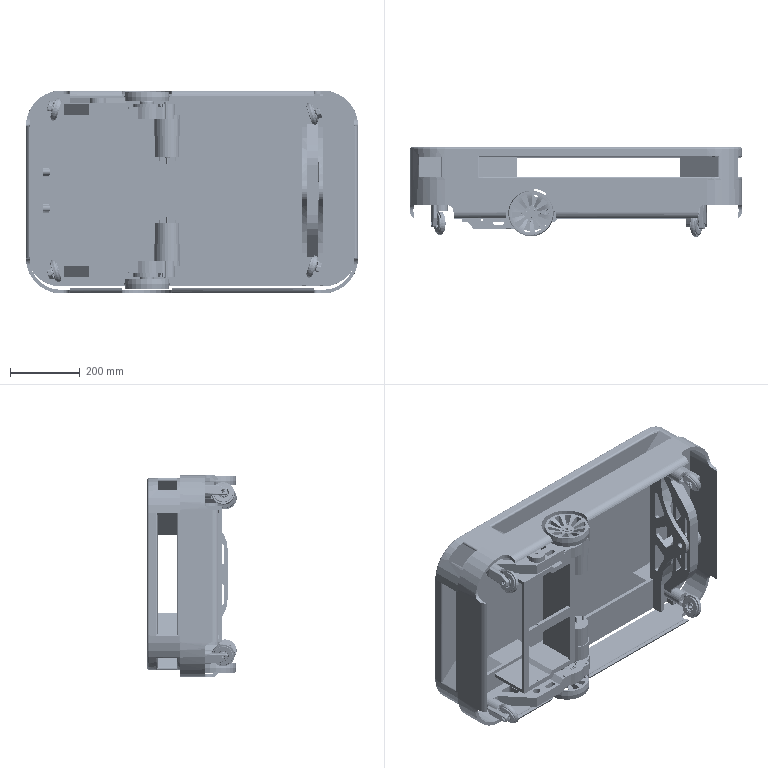Assembly | SolidWorks | mm | 60 component files | 355 solids | 6056 faces | box 950 x 255.66 x 580 mm | volume 29114725 mm3 | cylinder 3134 | plane 1494 | sphere 690 | torus 552 | cone 146 | spline 40 | commonest cylinder face diameters 1 x268 6.975 x266 0.6 x260 6.15 x192 23.75 x168 21.25 x168 4 x162 10 x133
Bill of materials:
Bracket1 | 1 |  | Elongated stepped bracket/plate. At one end is a rounded eye with a hexagonal hole. A triangular cutout and rectangular, round and slotted openings run along the body. At the other end is a large circular bore with a counterbored/recessed seat, an adjacent smaller round hole, and several small holes around both bores.
BrushedDCMotor | 1 |  | Cylindrical body with two diameters. A stepped shaft protrudes from one end face, which has a raised boss. A small offset feature and pin-like protrusions are at the opposite end.
DriveWheel | 1 |  | Wheel-like disc, or rim, with a flanged outer rim and twelve tapered radial spokes. The central hub opening has semicircular notches around it.
DriveWheelRubber | 1 | Natural Rubber | Thin-walled cylindrical ring or band with a short axial length relative to its diameter. The outer surface appears slightly crowned or faceted.
FlatWasher | 1 |  | Flat annular disc with a central circular hole: a plain washer-like shape.
Gasket | 4 |  | Flat open ring with a gap. Each end has a lug with a small hole. The shape resembles an internal-style retaining ring, with the lugs on the inner side.
GB_T276-2013[DeepGrooveBallBearing[60000]608] | 1 | AISI 304 | Annular assembly-like body: concentric outer and inner rings separated by a gap, with a central bore. The edges are rounded.
Gb_t276-2013[DeepGrooveBallBearing[60000]61908] | 2 |  | Thin-section annular body with concentric outer and inner rings, a narrow gap between them, and a large bore relative to its outer diameter.
GB_T276-2013[DeepGrooveBallBearing[60000]6300] | 7 | AISI 304 | Annular body with concentric outer and inner rings, an annular gap, and a relatively small central bore.
GuideWheelBracket | 2 |  | Arm or bracket with a cylindrical sleeve (a through-bore collar) at one end. A tapered flat lever extends from the sleeve to a rounded tip, which has a countersunk or counterbored small hole.
GuideWheelHub | 2 |  | Grooved ring, like a pulley or grommet: an annular body with a concave groove around its outside between two flanges, and a central bore with an internal step.
GuideWheelRubber | 2 |  | Annular ring with a roughly rectangular cross-section and slightly rounded edges. The section is thicker radially than the thin band part.
LargeGear | 1 |  | Compound spur-gear part: a thin wide toothed disc with a tall cylindrical hub on one face. A smaller lobed boss with six rounded lobes sits on top of the hub, and a small round bore runs through the center.
ProtectivePlate | 1 |  | Flat plate with a large circular through-opening and a smaller circular through-opening beside it. The outline is mostly rectangular, with arc-shaped bulges around both openings. There are four small corner holes, and part of the plate is a thicker raised region.
SmallGear | 1 |  | Spur gear with a short raised collar on one face. Its central bore is D-shaped, with one flat side.
DeepGrooveBallBearing[60000][61900] | 1 | AISI 304 | Ring assembly with concentric inner and outer rings and a visible annular gap between them, in a form that looks like a bearing. It is relatively wide compared with the ring cross-section.
GuideWheelBracket2 | 1 |  | Elongated bracket link with a curved, offset body. Each end has a rounded eye with a hexagonal hole. The central web has triangular and slot-shaped lightening cutouts arranged like a truss around a small round hole.
MirrorGasket | 4 |  | Thin flat open ring with a gap. Each end of the opening has a lug with a small round hole. The overall form resembles a retaining ring.
MirrorGB_T276-2013[DeepGrooveBallBearing[60000]6300] | 7 | AISI 304 | Ring assembly with concentric inner and outer rings and an annular gap between them, in a form that looks like a bearing. It has a smaller bore relative to its outer diameter than unnamed part.
MirrorGuideWheelBracket | 2 |  | Clamp-like arm: a cylindrical collar with a large bore, with a lever arm extending from one side. Near the end of the arm is a small round hole with a hexagonal recess.
MirrorGuideWheelHub | 2 |  | Grooved wheel or pulley-like ring: an annular body with a concave groove running around its outer edge between two flanges, and a large central bore.
MirrorGuideWheelRubber | 2 |  | Plain ring with a roughly rectangular cross-section, rounded or slightly chamfered edges, and a large inner diameter compared with its wall thickness.
MirrorBracket1 | 1 |  | Mounting-plate bracket with an irregular outline and a stepped thickness. It has a large circular opening and a smaller circular opening ringed by a pattern of small holes. There are also rectangular slots, a round hole, a triangular cutout, and an end eye with a hexagonal hole.
MirrorBrushedDCMotor | 1 |  | Cylindrical body made of two coaxial sections of slightly different diameters. One end has a small central shaft and two flat tab-like protrusions. The other end has an off-center smaller cylindrical boss and a stepped output shaft. The form resembles a geared-motor housing.
MirrorDriveWheel | 1 |  | Spoked wheel or spool-like disc. A circular body has twelve tapered spoke windows, a central bore with semicircular notches around it, and a raised flange at each axial end with a shallow recessed band between them.
MirrorDriveWheelRubber | 1 | Natural Rubber | Short thin-walled cylindrical ring (band) with an open bore and a small radial wall thickness. The outer surface has a slight break or taper at mid-height.
MirrorFlatWasher | 1 |  | Flat annular disc (washer-like) with one concentric through-hole and uniform thickness.
MirrorGB_T276-2013[DeepGrooveBallBearing[60000]608] | 1 | AISI 304 | Group of concentric rings: an outer ring and an inner ring with a central bore, separated by an annular gap that holds a thinner intermediate ring. The edges are rounded. The overall form looks like a bearing.
Mirrorgb_t276-2013[DeepGrooveBallBearing[60000]61908] | 2 |  | Thin-section set of concentric rings: an outer ring and an inner ring with a large bore, separated by a narrow gap. The edges are rounded. The form looks like a thin-section bearing.
MirrorGuardPlate | 1 |  | Stepped mounting plate (flange). It has a large circular through-opening with an internal step, a side lobe with a smaller stepped circular opening, and four corner through-holes in a rectangular plate region with rounded corners.
MirrorLargeGear | 1 |  | Compound spur gear part: a large spur gear ring around a tall cylindrical hub, with a smaller toothed pinion section at one end. There is a hexagonal recess at the top of the hub and a small round axial hole.
MirrorSmallGear | 1 |  | Spur gear with straight teeth, a central bore that appears to have one flat (D-shaped), and a short smaller-diameter hub shoulder on one face.
Part27 | 1 |  | Thin-walled rounded-rectangle frame (open band) with no top or bottom face. It has a semicircular notch in the edge of each long side and rectangular relief notches near the corners.
Tray | 1 |  | Complex shallow housing or tray: a rounded-rectangle body with a flat face plate, an internal perimeter frame and ribs, a box-like compartment near one end, curved slotted arm features near the other end, and small pins or tabs on the face.
Mates:
1. parallel | FrontGuideWheel-1/GuideWheelBracket2-1 face at (544.259, 72.387, -327.387) dir (0, 1, 0) | Tray-2 face at (-191.241, 138, -41.572) dir (0, -1, 0)
2. width | FrontGuideWheel-1/GuideWheelBracket2-1 face at (544.259, 87.387, -288.413) dir (1, 0, 0) | FrontGuideWheel-1/GuideWheelBracket2-1 face at (513.259, 87.387, -288.413) dir (-1, 0, 0) | Tray-2 face at (545.759, 3.167, 58.428) dir (-1, 0, 0) | Tray-2 face at (511.759, 3.167, 58.428) dir (1, 0, 0)
3. parallel | DriveDevice-1/Bracket1-1 face at (0, 0, 31) dir (0, 0, 1) | Tray-2 face at (558.759, 232, 58.428) dir (0, 0, 1)
4. distance | DriveDevice-1/Bracket1-1 face at (0, 118, 31) dir (0, 1, 0) | Tray-2 face at (-191.241, 138, -41.572) dir (0, -1, 0)
5. concentric | FrontGuideWheel-1/DeepGrooveBallBearing[60000][61900]-1 edge at (544.559, 27.686, -216.572) dir (-1, 0, 0) r 5.3 | Tray-2 edge at (558.759, 27.686, -216.572) dir (1, 0, 0) r 8.309
6. width | Tray-2 face at (498.759, 110, -486.572) dir (-1, 0, 0) | Tray-2 face at (558.759, 110, -486.572) dir (1, 0, 0) | FrontGuideWheel-1/GuideWheelBracket2-1 face at (544.259, 87.387, -288.413) dir (1, 0, 0) | FrontGuideWheel-1/GuideWheelBracket2-1 face at (513.259, 87.387, -288.413) dir (-1, 0, 0)
7. coincident | Tray-2 face at (-191.241, 138, -41.572) dir (0, -1, 0) | Part27-1 face at (-191.241, 138, -411.572) dir (0, 1, 0)
8. coincident | Tray-2 face at (-291.241, 232, -41.572) dir (-1, 0, 0) | Part27-1 face at (-291.241, 28, -31.572) dir (-1, 0, 0)
9. coincident | Tray-2 face at (558.759, 232, 58.428) dir (0, 0, 1) | Part27-1 face at (558.759, 28, 58.428) dir (0, 0, -1)
10. concentric | Bracket1-1 edge at (55, 43, 2.5) dir (0, 0, -1) r 32.2 | Gb_t276-2013[DeepGrooveBallBearing[60000]61908]-1 edge at (55, 43, -9.9) dir (0, 0, 1) r 31
11. coincident | Bracket1-1 face at (55, 43, -10.5) dir (0, 0, 1) | Gb_t276-2013[DeepGrooveBallBearing[60000]61908]-1 face at (71.985, 68.212, -10.5) dir (0, 0, -1)
12. concentric | Gb_t276-2013[DeepGrooveBallBearing[60000]61908]-1 edge at (55, 43, 1.5) dir (0, 0, 1) r 20.6 | LargeGear-1 edge at (55, 43, -13) dir (0, 0, -1) r 18.8
13. coincident | Gb_t276-2013[DeepGrooveBallBearing[60000]61908]-1 face at (66.51, 60.085, 1.5) dir (0, 0, 1) | LargeGear-1 face at (55, 43, 1.5) dir (0, 0, -1)
14. concentric | LargeGear-1 edge at (55, 43, 37.5) dir (0, 0, 1) r 18.8 | Gb_t276-2013[DeepGrooveBallBearing[60000]61908]-2 edge at (55, 43, 27.5) dir (0, 0, 1) r 20.6
15. coincident | LargeGear-1 face at (55, 43, 15.5) dir (0, 0, 1) | Gb_t276-2013[DeepGrooveBallBearing[60000]61908]-2 face at (73.287, 67.285, 15.5) dir (0, 0, -1)
16. coincident | Bracket1-1 face at (0, 0, 2.5) dir (0, 0, 1) | SmallGear-1 face at (109.394, 58.688, 2.5) dir (0, 0, -1)
17. coincident | SmallGear-1 face at (110, 43, 14.5) dir (0, 0, 1) | GB_T276-2013[DeepGrooveBallBearing[60000]6300]-1 face at (117.32, 58.232, 14.5) dir (0, 0, -1)
18. concentric | LargeGear-1 edge at (55, 43, 37.5) dir (0, 0, 1) r 18.8 | ProtectivePlate-1 edge at (55, 43, 31.5) dir (0, 0, 1) r 30.2
19. coincident | Bracket1-1 face at (0, 0, 16.5) dir (0, 0, 1) | ProtectivePlate-1 face at (85.418, 8.541, 16.5) dir (0, 0, -1)
20. concentric | LargeGear-1 edge at (55, 43, 53.5) dir (0, 0, 1) r 4.3 | FlatWasher-1 edge at (55, 43, 53.5) dir (0, 0, -1) r 4.3
21. coincident | LargeGear-1 face at (55, 43, 53.5) dir (0, 0, 1) | FlatWasher-1 face at (55, 43, 53.5) dir (0, 0, -1)
22. concentric | LargeGear-1 edge at (55, 43, 53.5) dir (0, 0, 1) r 4.3 | DriveWheel-1 edge at (55, 43, 37.5) dir (0, 0, 1) r 62
23. coincident | LargeGear-1 face at (55, 43, 37.5) dir (0, 0, 1) | DriveWheel-1 face at (55, 43, 37.5) dir (0, 0, -1)
24. concentric | LargeGear-1 face at (58.449, 57.598, 52.5) dir (0, 0, -1) r 785.398 | DriveWheel-1 face at (58.449, 57.598, 37.5) dir (0, 0, 1) r 5.5
25. concentric | GB_T276-2013[DeepGrooveBallBearing[60000]6300]-2 edge at (-203.866, 70.2, 20) dir (0, -1, 0) r 13.933 | GB_T276-2013[DeepGrooveBallBearing[60000]6300]-3 edge at (-203.866, 70.2, 20) dir (0, 1, 0) r 5.6
26. coincident | GB_T276-2013[DeepGrooveBallBearing[60000]6300]-2 face at (-220.649, 70.2, 18.017) dir (0, -1, 0) | GB_T276-2013[DeepGrooveBallBearing[60000]6300]-3 face at (-186.966, 70.2, 20.101) dir (0, 1, 0)
27. concentric | GuideWheelHub-1 edge at (-210.9, 15, 15.884) dir (-0.9559, 0, 0.2937) r 14 | GB_T276-2013[DeepGrooveBallBearing[60000]6300]-4 edge at (-210.9, 15, 15.884) dir (0.9559, 0, -0.2937) r 16.9
28. parallel | SmallGear-1 face at (115.607, 45.136, 30.54) dir (-0.9875, 0.1577, 0) | BrushedDCMotor-1 face at (118.289, 61.93, -4.54) dir (0.9875, -0.1577, 0)
29. concentric | DriveWheel-1 edge at (55, 43, 65.5) dir (0, 0, 1) r 62 | DriveWheelRubber-1 edge at (55, 43, 61.5) dir (0, 0, 1) r 60
30. coincident | DriveWheel-1 face at (69.254, 103.339, 41.5) dir (0, 0, 1) | DriveWheelRubber-1 face at (48.726, 102.671, 41.5) dir (0, 0, -1)
31. coincident | GuideWheelHub-1 edge at (-210.893, 15, 15.882) dir (-0.9559, 0, 0.2937) r 28 | GuideWheelRubber-1 edge at (-210.893, 15, 15.882) dir (-0.9559, 0, 0.2937) r 28
32. coincident | GuideWheelHub-1 face at (-212.348, 1.897, 11.172) dir (0.9559, 0, -0.2937) | GB_T276-2013[DeepGrooveBallBearing[60000]6300]-4 face at (-213.884, 1.495, 6.173) dir (-0.9559, 0, 0.2937)
33. concentric | GuideWheelHub-1 edge at (-198.473, 15, 12.066) dir (-0.9559, 0, 0.2937) r 17.5 | Gasket-2 edge at (-198.473, 15, 12.066) dir (0.9559, 0, -0.2937) r 18.3
34. coincident | GuideWheelHub-1 face at (-200.386, -2.315, 5.84) dir (-0.9559, 0, 0.2937) | Gasket-2 face at (-198.473, 15, 12.066) dir (0.9559, 0, -0.2937)
35. coincident | Bracket1-1 face at (0, 0, 31) dir (0, 0, 1) | GB_T276-2013[DeepGrooveBallBearing[60000]608]-1 face at (-85, 35.7, 31) dir (0, 0, 1)
36. coincident | Bracket1-1 face at (0, 86, 31) dir (0, -1, 0) | GuideWheelBracket-1 face at (-197.992, 86, 39.118) dir (0, 1, 0)
37. coincident | Bracket1-1 face at (0, 0, -13.5) dir (0, 0, -1) | BrushedDCMotor-1 face at (113.154, 62.75, -13.5) dir (0, 0, 1)
38. coincident | Bracket1-1 face at (0, 0, 31) dir (1, 0, 0) | ProtectivePlate-1 face at (0, 8.541, 31.5) dir (-1, 0, 0)
39. concentric | Bracket1-1 face at (-85, 25, 31) dir (0, 0, -1) r 11 | GB_T276-2013[DeepGrooveBallBearing[60000]608]-1 face at (-85, 25, 24) dir (0, 0, -1) r 11
40. concentric | Bracket1-1 face at (-203.866, 86, 20) dir (0, 1, 0) r 20 | GB_T276-2013[DeepGrooveBallBearing[60000]6300]-2 face at (-203.866, 72.2, 20) dir (0, -1, 0) r 17.5
41. concentric | Bracket1-1 face at (-203.866, 86, 20) dir (0, 1, 0) r 20 | GuideWheelBracket-1 face at (-203.866, 50, 20) dir (0, -1, 0) r 20
42. concentric | Bracket1-1 face at (55, 43, -10.5) dir (0, 0, -1) r 30.1 | Gb_t276-2013[DeepGrooveBallBearing[60000]61908]-1 face at (55, 43, -1) dir (0, 0, 1) r 20
43. concentric | SmallGear-1 face at (110, 43, -7.5) dir (0, 0, 1) r 6 | BrushedDCMotor-1 face at (110, 43, 35.5) dir (0, 0, -1) r 6
44. concentric | Bracket1-1 face at (110, 43, 2.5) dir (0, 0, 1) r 20.3 | SmallGear-1 face at (110, 43, 14.5) dir (0, 0, -1) r 11
45. concentric | SmallGear-1 face at (110, 43, -7.5) dir (0, 0, 1) r 6 | GB_T276-2013[DeepGrooveBallBearing[60000]6300]-1 face at (110, 43, 23.5) dir (0, 0, 1) r 5
46. concentric | Bracket1-1 face at (110, 43, -13.5) dir (0, 0, 1) r 12.3 | SmallGear-1 face at (110, 43, -7.5) dir (0, 0, 1) r 6
47. coincident | GuideWheelBracket2-1 face at (-190, 31, -78) dir (0, 0, 1) | GuideWheel-1/GuideWheelBracket-1 face at (-193.663, 21.816, -78) dir (0, 0, -1)
48. concentric | GuideWheelBracket2-1 edge at (-212.639, 15.5, -78) dir (0, 0, -1) r 20 | GuideWheel-1/GuideWheelBracket-1 edge at (-212.639, 15.5, -78) dir (0, 0, 1) r 20
49. coincident | GuideWheelBracket2-1 edge at (0, 31, -25.299) dir (0, 1, 0) r 11 | DeepGrooveBallBearing[60000][61900]-1 edge at (0, 31, -25.299) dir (0, -1, 0) r 11
50. parallel | GuideWheelBracket2-1 face at (71.841, 31, -85) dir (0, 1, 0) | DeepGrooveBallBearing[60000][61900]-1 face at (-9.638, 31.3, -29.947) dir (0, 1, 0)
51. concentric | GB_T276-2013[DeepGrooveBallBearing[60000]6300]-2 edge at (-203.866, 70.2, 20) dir (0, -1, 0) r 13.933 | GB_T276-2013[DeepGrooveBallBearing[60000]6300]-3 edge at (-203.866, 70.2, 20) dir (0, 1, 0) r 5.6
52. coincident | GB_T276-2013[DeepGrooveBallBearing[60000]6300]-2 face at (-220.649, 70.2, 18.017) dir (0, -1, 0) | GB_T276-2013[DeepGrooveBallBearing[60000]6300]-3 face at (-186.966, 70.2, 20.101) dir (0, 1, 0)
53. concentric | GuideWheelHub-1 edge at (-210.9, 15, 15.884) dir (-0.9559, 0, 0.2937) r 14 | GB_T276-2013[DeepGrooveBallBearing[60000]6300]-4 edge at (-210.9, 15, 15.884) dir (0.9559, 0, -0.2937) r 16.9
54. coincident | GuideWheelHub-1 edge at (-210.893, 15, 15.882) dir (-0.9559, 0, 0.2937) r 28 | GuideWheelRubber-1 edge at (-210.893, 15, 15.882) dir (-0.9559, 0, 0.2937) r 28
55. coincident | GuideWheelHub-1 face at (-212.348, 1.897, 11.172) dir (0.9559, 0, -0.2937) | GB_T276-2013[DeepGrooveBallBearing[60000]6300]-4 face at (-213.884, 1.495, 6.173) dir (-0.9559, 0, 0.2937)
56. concentric | GuideWheelHub-1 edge at (-198.473, 15, 12.066) dir (-0.9559, 0, 0.2937) r 17.5 | Gasket-2 edge at (-198.473, 15, 12.066) dir (0.9559, 0, -0.2937) r 18.3
57. coincident | GuideWheelHub-1 face at (-200.386, -2.315, 5.84) dir (-0.9559, 0, 0.2937) | Gasket-2 face at (-198.473, 15, 12.066) dir (0.9559, 0, -0.2937)